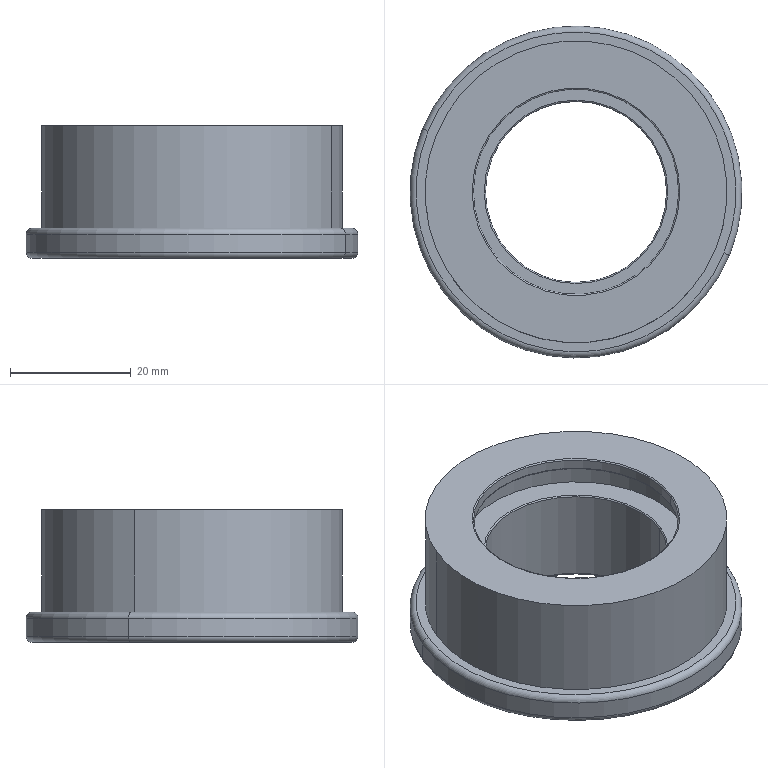Component | SolidWorks | Cylinder-1_GuideSleeve-1 | 1 solid | 27 faces | box 55 x 55 x 22 mm | volume 27518 mm3 | torus 12 | cylinder 10 | plane 5 | commonest cylinder face diameters 55 x2 50 x2 34 x2 38 x2 30 x2
build123d program:
from build123d import *

# Parameters (mm, degrees)
FILLET1_R = 1
FILLET2_R = 0.3
FILLET3_R = 0.2


with BuildPart() as part:
    # Sketch1 → Revolve1 (revolve)
    with BuildSketch(Plane.XY, mode=Mode.PRIVATE) as revolve1_sk:
        Polygon((0, 15), (16, 15), (16, 19), (20, 19), (20, 17), (22, 17), (22, 25), (5, 25), (5, 27.5), (0, 27.5), align=None)
    revolve(revolve1_sk.sketch.rotate(Axis((-21.725, 0, 0), (1, 0, 0)), 90), axis=Axis((-21.725, 0, 0), (1, 0, 0)))

    # Fillet1
    fillet1_edges = [part.edges().sort_by_distance(p)[0] for p in [
        (0, 0, -27.5),
        (5, 0, -27.5),
    ]]
    fillet(fillet1_edges, radius=FILLET1_R)

    # Fillet2
    fillet2_edges = [part.edges().sort_by_distance(p)[0] for p in [
        (0, 0, -15),
    ]]
    fillet(fillet2_edges, radius=FILLET2_R)

    # Fillet3
    fillet3_edges = [part.edges().sort_by_distance(p)[0] for p in [
        (16, 0, -15),
        (22, 0, -17),
        (20, 0, -17),
    ]]
    fillet(fillet3_edges, radius=FILLET3_R)


solid = part.part

# Placed as in the assembly
solid = solid.moved(Location((-180.557, 26.412, -199.351), (0, -90, 0)))
STEP:
#1=COLOUR_RGB('',0.7922,0.8196,0.9333);
#2=FILL_AREA_STYLE_COLOUR('',#1);
#3=FILL_AREA_STYLE('',(#2));
#4=SURFACE_STYLE_FILL_AREA(#3);
#5=SURFACE_SIDE_STYLE('',(#4));
#6=SURFACE_STYLE_USAGE(.BOTH.,#5);
#7=PRESENTATION_STYLE_ASSIGNMENT((#6));
#8=CARTESIAN_POINT('',(-6.563,0.8143,-7.226));
#9=VERTEX_POINT('',#8);
#10=CARTESIAN_POINT('',(-7.654,1.265,-7.226));
#11=VERTEX_POINT('',#10);
#12=CARTESIAN_POINT('',(-7.109,1.04,-7.226));
#13=DIRECTION('',(-0.,0.,1.));
#14=DIRECTION('',(-0.9242,0.3818,0.));
#15=AXIS2_PLACEMENT_3D('',#12,#13,#14);
#16=CIRCLE('',#15,0.5906);
#17=EDGE_CURVE('',#9,#11,#16,.T.);
#18=ORIENTED_EDGE('',*,*,#17,.F.);
#19=CARTESIAN_POINT('',(-6.555,0.8113,-7.219));
#20=VERTEX_POINT('',#19);
#21=CARTESIAN_POINT('',(-6.555,0.8113,-7.226));
#22=DIRECTION('',(0.3818,0.9242,-0.));
#23=DIRECTION('',(-0.9242,0.3818,0.));
#24=AXIS2_PLACEMENT_3D('',#21,#22,#23);
#25=CIRCLE('',#24,0.007874);
#26=EDGE_CURVE('',#9,#20,#25,.T.);
#27=ORIENTED_EDGE('',*,*,#26,.T.);
#28=CARTESIAN_POINT('',(-7.662,1.268,-7.219));
#29=VERTEX_POINT('',#28);
#30=CARTESIAN_POINT('',(-7.109,1.04,-7.219));
#31=DIRECTION('',(0.,-0.,-1.));
#32=DIRECTION('',(-0.9242,0.3818,0.));
#33=AXIS2_PLACEMENT_3D('',#30,#31,#32);
#34=CIRCLE('',#33,0.5984);
#35=EDGE_CURVE('',#29,#20,#34,.T.);
#36=ORIENTED_EDGE('',*,*,#35,.F.);
#37=CARTESIAN_POINT('',(-7.662,1.268,-7.226));
#38=DIRECTION('',(-0.3818,-0.9242,0.));
#39=DIRECTION('',(0.9242,-0.3818,0.));
#40=AXIS2_PLACEMENT_3D('',#37,#38,#39);
#41=CIRCLE('',#40,0.007874);
#42=EDGE_CURVE('',#11,#29,#41,.T.);
#43=ORIENTED_EDGE('',*,*,#42,.F.);
#44=EDGE_LOOP('',(#18,#27,#36,#43));
#45=FACE_OUTER_BOUND('',#44,.T.);
#46=CARTESIAN_POINT('',(-7.109,1.04,-7.226));
#47=DIRECTION('',(0.,-0.,-1.));
#48=DIRECTION('',(-0.9242,0.3818,-0.));
#49=AXIS2_PLACEMENT_3D('',#46,#47,#48);
#50=TOROIDAL_SURFACE('',#49,0.5984,0.007874);
#51=ADVANCED_FACE('',(#45),#50,.T.);
#52=CARTESIAN_POINT('',(-7.727,1.295,-7.053));
#53=VERTEX_POINT('',#52);
#54=CARTESIAN_POINT('',(-6.49,0.7843,-7.053));
#55=VERTEX_POINT('',#54);
#56=CARTESIAN_POINT('',(-7.109,1.04,-7.053));
#57=DIRECTION('',(0.,-0.,-1.));
#58=DIRECTION('',(0.9242,-0.3818,0.));
#59=AXIS2_PLACEMENT_3D('',#56,#57,#58);
#60=CIRCLE('',#59,0.6693);
#61=EDGE_CURVE('',#53,#55,#60,.T.);
#62=ORIENTED_EDGE('',*,*,#61,.F.);
#63=CARTESIAN_POINT('',(-7.734,1.298,-7.061));
#64=VERTEX_POINT('',#63);
#65=CARTESIAN_POINT('',(-7.734,1.298,-7.053));
#66=DIRECTION('',(0.3818,0.9242,-0.));
#67=DIRECTION('',(-0.9242,0.3818,0.));
#68=AXIS2_PLACEMENT_3D('',#65,#66,#67);
#69=CIRCLE('',#68,0.007874);
#70=EDGE_CURVE('',#53,#64,#69,.T.);
#71=ORIENTED_EDGE('',*,*,#70,.T.);
#72=CARTESIAN_POINT('',(-6.483,0.7813,-7.061));
#73=VERTEX_POINT('',#72);
#74=CARTESIAN_POINT('',(-7.109,1.04,-7.061));
#75=DIRECTION('',(-0.,0.,1.));
#76=DIRECTION('',(0.9242,-0.3818,0.));
#77=AXIS2_PLACEMENT_3D('',#74,#75,#76);
#78=CIRCLE('',#77,0.6772);
#79=EDGE_CURVE('',#73,#64,#78,.T.);
#80=ORIENTED_EDGE('',*,*,#79,.F.);
#81=CARTESIAN_POINT('',(-6.483,0.7813,-7.053));
#82=DIRECTION('',(-0.3818,-0.9242,0.));
#83=DIRECTION('',(0.9242,-0.3818,0.));
#84=AXIS2_PLACEMENT_3D('',#81,#82,#83);
#85=CIRCLE('',#84,0.007874);
#86=EDGE_CURVE('',#55,#73,#85,.T.);
#87=ORIENTED_EDGE('',*,*,#86,.F.);
#88=EDGE_LOOP('',(#62,#71,#80,#87));
#89=FACE_OUTER_BOUND('',#88,.T.);
#90=CARTESIAN_POINT('',(-7.109,1.04,-7.053));
#91=DIRECTION('',(-0.,0.,1.));
#92=DIRECTION('',(0.9242,-0.3818,0.));
#93=AXIS2_PLACEMENT_3D('',#90,#91,#92);
#94=TOROIDAL_SURFACE('',#93,0.6772,0.007874);
#95=ADVANCED_FACE('',(#89),#94,.T.);
#96=CARTESIAN_POINT('',(-6.49,0.7843,-6.99));
#97=VERTEX_POINT('',#96);
#98=CARTESIAN_POINT('',(-7.727,1.295,-6.99));
#99=VERTEX_POINT('',#98);
#100=CARTESIAN_POINT('',(-7.109,1.04,-6.99));
#101=DIRECTION('',(-0.,0.,1.));
#102=DIRECTION('',(-0.9242,0.3818,0.));
#103=AXIS2_PLACEMENT_3D('',#100,#101,#102);
#104=CIRCLE('',#103,0.6693);
#105=EDGE_CURVE('',#97,#99,#104,.T.);
#106=ORIENTED_EDGE('',*,*,#105,.F.);
#107=CARTESIAN_POINT('',(-6.483,0.7813,-6.982));
#108=VERTEX_POINT('',#107);
#109=CARTESIAN_POINT('',(-6.483,0.7813,-6.99));
#110=DIRECTION('',(0.3818,0.9242,-0.));
#111=DIRECTION('',(-0.9242,0.3818,0.));
#112=AXIS2_PLACEMENT_3D('',#109,#110,#111);
#113=CIRCLE('',#112,0.007874);
#114=EDGE_CURVE('',#97,#108,#113,.T.);
#115=ORIENTED_EDGE('',*,*,#114,.T.);
#116=CARTESIAN_POINT('',(-7.734,1.298,-6.982));
#117=VERTEX_POINT('',#116);
#118=CARTESIAN_POINT('',(-7.109,1.04,-6.982));
#119=DIRECTION('',(0.,-0.,-1.));
#120=DIRECTION('',(-0.9242,0.3818,0.));
#121=AXIS2_PLACEMENT_3D('',#118,#119,#120);
#122=CIRCLE('',#121,0.6772);
#123=EDGE_CURVE('',#117,#108,#122,.T.);
#124=ORIENTED_EDGE('',*,*,#123,.F.);
#125=CARTESIAN_POINT('',(-7.734,1.298,-6.99));
#126=DIRECTION('',(-0.3818,-0.9242,0.));
#127=DIRECTION('',(0.9242,-0.3818,0.));
#128=AXIS2_PLACEMENT_3D('',#125,#126,#127);
#129=CIRCLE('',#128,0.007874);
#130=EDGE_CURVE('',#99,#117,#129,.T.);
#131=ORIENTED_EDGE('',*,*,#130,.F.);
#132=EDGE_LOOP('',(#106,#115,#124,#131));
#133=FACE_OUTER_BOUND('',#132,.T.);
#134=CARTESIAN_POINT('',(-7.109,1.04,-6.99));
#135=DIRECTION('',(0.,-0.,-1.));
#136=DIRECTION('',(-0.9242,0.3818,-0.));
#137=AXIS2_PLACEMENT_3D('',#134,#135,#136);
#138=TOROIDAL_SURFACE('',#137,0.6772,0.007874);
#139=ADVANCED_FACE('',(#133),#138,.T.);
#140=CARTESIAN_POINT('',(-7.654,1.265,-7.837));
#141=VERTEX_POINT('',#140);
#142=CARTESIAN_POINT('',(-6.563,0.8143,-7.837));
#143=VERTEX_POINT('',#142);
#144=CARTESIAN_POINT('',(-7.109,1.04,-7.837));
#145=DIRECTION('',(0.,-0.,-1.));
#146=DIRECTION('',(0.9242,-0.3818,0.));
#147=AXIS2_PLACEMENT_3D('',#144,#145,#146);
#148=CIRCLE('',#147,0.5906);
#149=EDGE_CURVE('',#141,#143,#148,.T.);
#150=ORIENTED_EDGE('',*,*,#149,.F.);
#151=CARTESIAN_POINT('',(-7.665,1.27,-7.848));
#152=VERTEX_POINT('',#151);
#153=CARTESIAN_POINT('',(-7.665,1.27,-7.837));
#154=DIRECTION('',(0.3818,0.9242,-0.));
#155=DIRECTION('',(-0.9242,0.3818,0.));
#156=AXIS2_PLACEMENT_3D('',#153,#154,#155);
#157=CIRCLE('',#156,0.01181);
#158=EDGE_CURVE('',#141,#152,#157,.T.);
#159=ORIENTED_EDGE('',*,*,#158,.T.);
#160=CARTESIAN_POINT('',(-6.552,0.8098,-7.848));
#161=VERTEX_POINT('',#160);
#162=CARTESIAN_POINT('',(-7.109,1.04,-7.848));
#163=DIRECTION('',(-0.,0.,1.));
#164=DIRECTION('',(0.9242,-0.3818,0.));
#165=AXIS2_PLACEMENT_3D('',#162,#163,#164);
#166=CIRCLE('',#165,0.6024);
#167=EDGE_CURVE('',#161,#152,#166,.T.);
#168=ORIENTED_EDGE('',*,*,#167,.F.);
#169=CARTESIAN_POINT('',(-6.552,0.8098,-7.837));
#170=DIRECTION('',(-0.3818,-0.9242,0.));
#171=DIRECTION('',(0.9242,-0.3818,0.));
#172=AXIS2_PLACEMENT_3D('',#169,#170,#171);
#173=CIRCLE('',#172,0.01181);
#174=EDGE_CURVE('',#143,#161,#173,.T.);
#175=ORIENTED_EDGE('',*,*,#174,.F.);
#176=EDGE_LOOP('',(#150,#159,#168,#175));
#177=FACE_OUTER_BOUND('',#176,.T.);
#178=CARTESIAN_POINT('',(-7.109,1.04,-7.837));
#179=DIRECTION('',(-0.,0.,1.));
#180=DIRECTION('',(0.9242,-0.3818,0.));
#181=AXIS2_PLACEMENT_3D('',#178,#179,#180);
#182=TOROIDAL_SURFACE('',#181,0.6024,0.01181);
#183=ADVANCED_FACE('',(#177),#182,.T.);
#184=CARTESIAN_POINT('',(-6.144,0.6415,-7.652));
#185=VERTEX_POINT('',#184);
#186=CARTESIAN_POINT('',(-8.073,1.438,-7.652));
#187=VERTEX_POINT('',#186);
#188=CARTESIAN_POINT('',(-7.109,1.04,-7.652));
#189=DIRECTION('',(-0.,0.,1.));
#190=DIRECTION('',(-0.9242,0.3818,0.));
#191=AXIS2_PLACEMENT_3D('',#188,#189,#190);
#192=CIRCLE('',#191,1.043);
#193=EDGE_CURVE('',#185,#187,#192,.T.);
#194=ORIENTED_EDGE('',*,*,#193,.F.);
#195=CARTESIAN_POINT('',(-6.108,0.6264,-7.691));
#196=VERTEX_POINT('',#195);
#197=CARTESIAN_POINT('',(-6.144,0.6415,-7.691));
#198=DIRECTION('',(0.3818,0.9242,-0.));
#199=DIRECTION('',(-0.9242,0.3818,0.));
#200=AXIS2_PLACEMENT_3D('',#197,#198,#199);
#201=CIRCLE('',#200,0.03937);
#202=EDGE_CURVE('',#185,#196,#201,.T.);
#203=ORIENTED_EDGE('',*,*,#202,.T.);
#204=CARTESIAN_POINT('',(-8.109,1.453,-7.691));
#205=VERTEX_POINT('',#204);
#206=CARTESIAN_POINT('',(-7.109,1.04,-7.691));
#207=DIRECTION('',(0.,-0.,-1.));
#208=DIRECTION('',(-0.9242,0.3818,0.));
#209=AXIS2_PLACEMENT_3D('',#206,#207,#208);
#210=CIRCLE('',#209,1.083);
#211=EDGE_CURVE('',#205,#196,#210,.T.);
#212=ORIENTED_EDGE('',*,*,#211,.F.);
#213=CARTESIAN_POINT('',(-8.073,1.438,-7.691));
#214=DIRECTION('',(-0.3818,-0.9242,0.));
#215=DIRECTION('',(0.9242,-0.3818,0.));
#216=AXIS2_PLACEMENT_3D('',#213,#214,#215);
#217=CIRCLE('',#216,0.03937);
#218=EDGE_CURVE('',#187,#205,#217,.T.);
#219=ORIENTED_EDGE('',*,*,#218,.F.);
#220=EDGE_LOOP('',(#194,#203,#212,#219));
#221=FACE_OUTER_BOUND('',#220,.T.);
#222=CARTESIAN_POINT('',(-7.109,1.04,-7.691));
#223=DIRECTION('',(0.,-0.,-1.));
#224=DIRECTION('',(-0.9242,0.3818,-0.));
#225=AXIS2_PLACEMENT_3D('',#222,#223,#224);
#226=TOROIDAL_SURFACE('',#225,1.043,0.03937);
#227=ADVANCED_FACE('',(#221),#226,.T.);
#228=CARTESIAN_POINT('',(-8.073,1.438,-7.848));
#229=VERTEX_POINT('',#228);
#230=CARTESIAN_POINT('',(-6.144,0.6415,-7.848));
#231=VERTEX_POINT('',#230);
#232=CARTESIAN_POINT('',(-7.109,1.04,-7.848));
#233=DIRECTION('',(0.,-0.,-1.));
#234=DIRECTION('',(0.9242,-0.3818,0.));
#235=AXIS2_PLACEMENT_3D('',#232,#233,#234);
#236=CIRCLE('',#235,1.043);
#237=EDGE_CURVE('',#229,#231,#236,.T.);
#238=ORIENTED_EDGE('',*,*,#237,.F.);
#239=CARTESIAN_POINT('',(-8.109,1.453,-7.809));
#240=VERTEX_POINT('',#239);
#241=CARTESIAN_POINT('',(-8.073,1.438,-7.809));
#242=DIRECTION('',(0.3818,0.9242,-0.));
#243=DIRECTION('',(-0.9242,0.3818,0.));
#244=AXIS2_PLACEMENT_3D('',#241,#242,#243);
#245=CIRCLE('',#244,0.03937);
#246=EDGE_CURVE('',#229,#240,#245,.T.);
#247=ORIENTED_EDGE('',*,*,#246,.T.);
#248=CARTESIAN_POINT('',(-6.108,0.6264,-7.809));
#249=VERTEX_POINT('',#248);
#250=CARTESIAN_POINT('',(-7.109,1.04,-7.809));
#251=DIRECTION('',(-0.,0.,1.));
#252=DIRECTION('',(0.9242,-0.3818,0.));
#253=AXIS2_PLACEMENT_3D('',#250,#251,#252);
#254=CIRCLE('',#253,1.083);
#255=EDGE_CURVE('',#249,#240,#254,.T.);
#256=ORIENTED_EDGE('',*,*,#255,.F.);
#257=CARTESIAN_POINT('',(-6.144,0.6415,-7.809));
#258=DIRECTION('',(-0.3818,-0.9242,0.));
#259=DIRECTION('',(0.9242,-0.3818,0.));
#260=AXIS2_PLACEMENT_3D('',#257,#258,#259);
#261=CIRCLE('',#260,0.03937);
#262=EDGE_CURVE('',#231,#249,#261,.T.);
#263=ORIENTED_EDGE('',*,*,#262,.F.);
#264=EDGE_LOOP('',(#238,#247,#256,#263));
#265=FACE_OUTER_BOUND('',#264,.T.);
#266=CARTESIAN_POINT('',(-7.109,1.04,-7.809));
#267=DIRECTION('',(-0.,0.,1.));
#268=DIRECTION('',(0.9242,-0.3818,0.));
#269=AXIS2_PLACEMENT_3D('',#266,#267,#268);
#270=TOROIDAL_SURFACE('',#269,1.043,0.03937);
#271=ADVANCED_FACE('',(#265),#270,.T.);
#272=ORIENTED_EDGE('',*,*,#211,.T.);
#273=CARTESIAN_POINT('',(-6.108,0.6264,-8.704));
#274=DIRECTION('',(0.,-0.,-1.));
#275=VECTOR('',#274,39.37);
#276=LINE('',#273,#275);
#277=EDGE_CURVE('',#196,#249,#276,.T.);
#278=ORIENTED_EDGE('',*,*,#277,.T.);
#279=ORIENTED_EDGE('',*,*,#255,.T.);
#280=CARTESIAN_POINT('',(-8.109,1.453,-8.704));
#281=DIRECTION('',(0.,-0.,-1.));
#282=VECTOR('',#281,39.37);
#283=LINE('',#280,#282);
#284=EDGE_CURVE('',#205,#240,#283,.T.);
#285=ORIENTED_EDGE('',*,*,#284,.F.);
#286=EDGE_LOOP('',(#272,#278,#279,#285));
#287=FACE_OUTER_BOUND('',#286,.T.);
#288=CARTESIAN_POINT('',(-7.109,1.04,-8.704));
#289=DIRECTION('',(0.,-0.,-1.));
#290=DIRECTION('',(-0.9242,0.3818,0.));
#291=AXIS2_PLACEMENT_3D('',#288,#289,#290);
#292=CYLINDRICAL_SURFACE('',#291,1.083);
#293=ADVANCED_FACE('',(#287),#292,.T.);
#294=CARTESIAN_POINT('',(-8.018,1.416,-6.982));
#295=VERTEX_POINT('',#294);
#296=CARTESIAN_POINT('',(-6.199,0.664,-6.982));
#297=VERTEX_POINT('',#296);
#298=CARTESIAN_POINT('',(-7.109,1.04,-6.982));
#299=DIRECTION('',(0.,-0.,-1.));
#300=DIRECTION('',(-0.9242,0.3818,0.));
#301=AXIS2_PLACEMENT_3D('',#298,#299,#300);
#302=CIRCLE('',#301,0.9843);
#303=EDGE_CURVE('',#295,#297,#302,.T.);
#304=ORIENTED_EDGE('',*,*,#303,.T.);
#305=CARTESIAN_POINT('',(-6.199,0.664,-7.652));
#306=VERTEX_POINT('',#305);
#307=CARTESIAN_POINT('',(-6.199,0.664,-8.704));
#308=DIRECTION('',(0.,-0.,-1.));
#309=VECTOR('',#308,39.37);
#310=LINE('',#307,#309);
#311=EDGE_CURVE('',#297,#306,#310,.T.);
#312=ORIENTED_EDGE('',*,*,#311,.T.);
#313=CARTESIAN_POINT('',(-8.018,1.416,-7.652));
#314=VERTEX_POINT('',#313);
#315=CARTESIAN_POINT('',(-7.109,1.04,-7.652));
#316=DIRECTION('',(0.,-0.,-1.));
#317=DIRECTION('',(-0.9242,0.3818,0.));
#318=AXIS2_PLACEMENT_3D('',#315,#316,#317);
#319=CIRCLE('',#318,0.9843);
#320=EDGE_CURVE('',#314,#306,#319,.T.);
#321=ORIENTED_EDGE('',*,*,#320,.F.);
#322=CARTESIAN_POINT('',(-8.018,1.416,-8.704));
#323=DIRECTION('',(0.,-0.,-1.));
#324=VECTOR('',#323,39.37);
#325=LINE('',#322,#324);
#326=EDGE_CURVE('',#295,#314,#325,.T.);
#327=ORIENTED_EDGE('',*,*,#326,.F.);
#328=EDGE_LOOP('',(#304,#312,#321,#327));
#329=FACE_OUTER_BOUND('',#328,.T.);
#330=CARTESIAN_POINT('',(-7.109,1.04,-8.704));
#331=DIRECTION('',(0.,-0.,-1.));
#332=DIRECTION('',(-0.9242,0.3818,0.));
#333=AXIS2_PLACEMENT_3D('',#330,#331,#332);
#334=CYLINDRICAL_SURFACE('',#333,0.9843);
#335=ADVANCED_FACE('',(#329),#334,.T.);
#336=CARTESIAN_POINT('',(-7.109,1.04,-6.99));
#337=DIRECTION('',(-0.,0.,1.));
#338=DIRECTION('',(-0.9242,0.3818,0.));
#339=AXIS2_PLACEMENT_3D('',#336,#337,#338);
#340=CIRCLE('',#339,0.6693);
#341=EDGE_CURVE('',#99,#97,#340,.T.);
#342=ORIENTED_EDGE('',*,*,#341,.T.);
#343=CARTESIAN_POINT('',(-6.49,0.7843,-8.704));
#344=DIRECTION('',(0.,-0.,-1.));
#345=VECTOR('',#344,39.37);
#346=LINE('',#343,#345);
#347=EDGE_CURVE('',#97,#55,#346,.T.);
#348=ORIENTED_EDGE('',*,*,#347,.T.);
#349=CARTESIAN_POINT('',(-7.109,1.04,-7.053));
#350=DIRECTION('',(0.,-0.,-1.));
#351=DIRECTION('',(0.9242,-0.3818,0.));
#352=AXIS2_PLACEMENT_3D('',#349,#350,#351);
#353=CIRCLE('',#352,0.6693);
#354=EDGE_CURVE('',#55,#53,#353,.T.);
#355=ORIENTED_EDGE('',*,*,#354,.T.);
#356=CARTESIAN_POINT('',(-7.727,1.295,-8.704));
#357=DIRECTION('',(0.,-0.,-1.));
#358=VECTOR('',#357,39.37);
#359=LINE('',#356,#358);
#360=EDGE_CURVE('',#99,#53,#359,.T.);
#361=ORIENTED_EDGE('',*,*,#360,.F.);
#362=EDGE_LOOP('',(#342,#348,#355,#361));
#363=FACE_OUTER_BOUND('',#362,.T.);
#364=CARTESIAN_POINT('',(-7.109,1.04,-8.704));
#365=DIRECTION('',(0.,-0.,-1.));
#366=DIRECTION('',(-0.9242,0.3818,0.));
#367=AXIS2_PLACEMENT_3D('',#364,#365,#366);
#368=CYLINDRICAL_SURFACE('',#367,0.6693);
#369=ADVANCED_FACE('',(#363),#368,.F.);
#370=CARTESIAN_POINT('',(-6.417,0.7542,-7.061));
#371=VERTEX_POINT('',#370);
#372=CARTESIAN_POINT('',(-7.8,1.325,-7.061));
#373=VERTEX_POINT('',#372);
#374=CARTESIAN_POINT('',(-7.109,1.04,-7.061));
#375=DIRECTION('',(0.,-0.,-1.));
#376=DIRECTION('',(-0.9242,0.3818,0.));
#377=AXIS2_PLACEMENT_3D('',#374,#375,#376);
#378=CIRCLE('',#377,0.748);
#379=EDGE_CURVE('',#371,#373,#378,.T.);
#380=ORIENTED_EDGE('',*,*,#379,.F.);
#381=CARTESIAN_POINT('',(-6.417,0.7542,-7.219));
#382=VERTEX_POINT('',#381);
#383=CARTESIAN_POINT('',(-6.417,0.7542,-8.704));
#384=DIRECTION('',(0.,-0.,-1.));
#385=VECTOR('',#384,39.37);
#386=LINE('',#383,#385);
#387=EDGE_CURVE('',#371,#382,#386,.T.);
#388=ORIENTED_EDGE('',*,*,#387,.T.);
#389=CARTESIAN_POINT('',(-7.8,1.325,-7.219));
#390=VERTEX_POINT('',#389);
#391=CARTESIAN_POINT('',(-7.109,1.04,-7.219));
#392=DIRECTION('',(0.,-0.,-1.));
#393=DIRECTION('',(-0.9242,0.3818,0.));
#394=AXIS2_PLACEMENT_3D('',#391,#392,#393);
#395=CIRCLE('',#394,0.748);
#396=EDGE_CURVE('',#382,#390,#395,.T.);
#397=ORIENTED_EDGE('',*,*,#396,.T.);
#398=CARTESIAN_POINT('',(-7.8,1.325,-8.704));
#399=DIRECTION('',(0.,-0.,-1.));
#400=VECTOR('',#399,39.37);
#401=LINE('',#398,#400);
#402=EDGE_CURVE('',#373,#390,#401,.T.);
#403=ORIENTED_EDGE('',*,*,#402,.F.);
#404=EDGE_LOOP('',(#380,#388,#397,#403));
#405=FACE_OUTER_BOUND('',#404,.T.);
#406=CARTESIAN_POINT('',(-7.109,1.04,-8.704));
#407=DIRECTION('',(0.,-0.,-1.));
#408=DIRECTION('',(-0.9242,0.3818,0.));
#409=AXIS2_PLACEMENT_3D('',#406,#407,#408);
#410=CYLINDRICAL_SURFACE('',#409,0.748);
#411=ADVANCED_FACE('',(#405),#410,.F.);
#412=CARTESIAN_POINT('',(-7.109,1.04,-7.226));
#413=DIRECTION('',(-0.,0.,1.));
#414=DIRECTION('',(-0.9242,0.3818,0.));
#415=AXIS2_PLACEMENT_3D('',#412,#413,#414);
#416=CIRCLE('',#415,0.5906);
#417=EDGE_CURVE('',#11,#9,#416,.T.);
#418=ORIENTED_EDGE('',*,*,#417,.T.);
#419=CARTESIAN_POINT('',(-6.563,0.8143,-8.704));
#420=DIRECTION('',(0.,-0.,-1.));
#421=VECTOR('',#420,39.37);
#422=LINE('',#419,#421);
#423=EDGE_CURVE('',#9,#143,#422,.T.);
#424=ORIENTED_EDGE('',*,*,#423,.T.);
#425=CARTESIAN_POINT('',(-7.109,1.04,-7.837));
#426=DIRECTION('',(0.,-0.,-1.));
#427=DIRECTION('',(0.9242,-0.3818,0.));
#428=AXIS2_PLACEMENT_3D('',#425,#426,#427);
#429=CIRCLE('',#428,0.5906);
#430=EDGE_CURVE('',#143,#141,#429,.T.);
#431=ORIENTED_EDGE('',*,*,#430,.T.);
#432=CARTESIAN_POINT('',(-7.654,1.265,-8.704));
#433=DIRECTION('',(0.,-0.,-1.));
#434=VECTOR('',#433,39.37);
#435=LINE('',#432,#434);
#436=EDGE_CURVE('',#11,#141,#435,.T.);
#437=ORIENTED_EDGE('',*,*,#436,.F.);
#438=EDGE_LOOP('',(#418,#424,#431,#437));
#439=FACE_OUTER_BOUND('',#438,.T.);
#440=CARTESIAN_POINT('',(-7.109,1.04,-8.704));
#441=DIRECTION('',(0.,-0.,-1.));
#442=DIRECTION('',(-0.9242,0.3818,0.));
#443=AXIS2_PLACEMENT_3D('',#440,#441,#442);
#444=CYLINDRICAL_SURFACE('',#443,0.5906);
#445=ADVANCED_FACE('',(#439),#444,.F.);
#446=ORIENTED_EDGE('',*,*,#167,.T.);
#447=CARTESIAN_POINT('',(-7.109,1.04,-7.848));
#448=DIRECTION('',(-0.,0.,1.));
#449=DIRECTION('',(0.9242,-0.3818,0.));
#450=AXIS2_PLACEMENT_3D('',#447,#448,#449);
#451=CIRCLE('',#450,0.6024);
#452=EDGE_CURVE('',#152,#161,#451,.T.);
#453=ORIENTED_EDGE('',*,*,#452,.T.);
#454=EDGE_LOOP('',(#446,#453));
#455=FACE_BOUND('',#454,.T.);
#456=CARTESIAN_POINT('',(-7.109,1.04,-7.848));
#457=DIRECTION('',(0.,-0.,-1.));
#458=DIRECTION('',(0.9242,-0.3818,0.));
#459=AXIS2_PLACEMENT_3D('',#456,#457,#458);
#460=CIRCLE('',#459,1.043);
#461=EDGE_CURVE('',#231,#229,#460,.T.);
#462=ORIENTED_EDGE('',*,*,#461,.T.);
#463=ORIENTED_EDGE('',*,*,#237,.T.);
#464=EDGE_LOOP('',(#462,#463));
#465=FACE_OUTER_BOUND('',#464,.T.);
#466=CARTESIAN_POINT('',(-6.695,2.04,-7.848));
#467=DIRECTION('',(-0.,0.,1.));
#468=DIRECTION('',(0.9242,-0.3818,0.));
#469=AXIS2_PLACEMENT_3D('',#466,#467,#468);
#470=PLANE('',#469);
#471=ADVANCED_FACE('',(#455,#465),#470,.F.);
#472=ORIENTED_EDGE('',*,*,#423,.F.);
#473=ORIENTED_EDGE('',*,*,#17,.T.);
#474=ORIENTED_EDGE('',*,*,#436,.T.);
#475=ORIENTED_EDGE('',*,*,#149,.T.);
#476=EDGE_LOOP('',(#472,#473,#474,#475));
#477=FACE_OUTER_BOUND('',#476,.T.);
#478=CARTESIAN_POINT('',(-7.109,1.04,-8.704));
#479=DIRECTION('',(0.,-0.,-1.));
#480=DIRECTION('',(-0.9242,0.3818,0.));
#481=AXIS2_PLACEMENT_3D('',#478,#479,#480);
#482=CYLINDRICAL_SURFACE('',#481,0.5906);
#483=ADVANCED_FACE('',(#477),#482,.F.);
#484=ORIENTED_EDGE('',*,*,#35,.T.);
#485=CARTESIAN_POINT('',(-7.109,1.04,-7.219));
#486=DIRECTION('',(0.,-0.,-1.));
#487=DIRECTION('',(-0.9242,0.3818,0.));
#488=AXIS2_PLACEMENT_3D('',#485,#486,#487);
#489=CIRCLE('',#488,0.5984);
#490=EDGE_CURVE('',#20,#29,#489,.T.);
#491=ORIENTED_EDGE('',*,*,#490,.T.);
#492=EDGE_LOOP('',(#484,#491));
#493=FACE_BOUND('',#492,.T.);
#494=CARTESIAN_POINT('',(-7.109,1.04,-7.219));
#495=DIRECTION('',(0.,-0.,-1.));
#496=DIRECTION('',(-0.9242,0.3818,0.));
#497=AXIS2_PLACEMENT_3D('',#494,#495,#496);
#498=CIRCLE('',#497,0.748);
#499=EDGE_CURVE('',#390,#382,#498,.T.);
#500=ORIENTED_EDGE('',*,*,#499,.F.);
#501=ORIENTED_EDGE('',*,*,#396,.F.);
#502=EDGE_LOOP('',(#500,#501));
#503=FACE_OUTER_BOUND('',#502,.T.);
#504=CARTESIAN_POINT('',(-6.883,1.586,-7.219));
#505=DIRECTION('',(0.,-0.,-1.));
#506=DIRECTION('',(-0.9242,0.3818,-0.));
#507=AXIS2_PLACEMENT_3D('',#504,#505,#506);
#508=PLANE('',#507);
#509=ADVANCED_FACE('',(#493,#503),#508,.F.);
#510=ORIENTED_EDGE('',*,*,#387,.F.);
#511=CARTESIAN_POINT('',(-7.109,1.04,-7.061));
#512=DIRECTION('',(0.,-0.,-1.));
#513=DIRECTION('',(-0.9242,0.3818,0.));
#514=AXIS2_PLACEMENT_3D('',#511,#512,#513);
#515=CIRCLE('',#514,0.748);
#516=EDGE_CURVE('',#373,#371,#515,.T.);
#517=ORIENTED_EDGE('',*,*,#516,.F.);
#518=ORIENTED_EDGE('',*,*,#402,.T.);
#519=ORIENTED_EDGE('',*,*,#499,.T.);
#520=EDGE_LOOP('',(#510,#517,#518,#519));
#521=FACE_OUTER_BOUND('',#520,.T.);
#522=CARTESIAN_POINT('',(-7.109,1.04,-8.704));
#523=DIRECTION('',(0.,-0.,-1.));
#524=DIRECTION('',(-0.9242,0.3818,0.));
#525=AXIS2_PLACEMENT_3D('',#522,#523,#524);
#526=CYLINDRICAL_SURFACE('',#525,0.748);
#527=ADVANCED_FACE('',(#521),#526,.F.);
#528=ORIENTED_EDGE('',*,*,#79,.T.);
#529=CARTESIAN_POINT('',(-7.109,1.04,-7.061));
#530=DIRECTION('',(-0.,0.,1.));
#531=DIRECTION('',(0.9242,-0.3818,0.));
#532=AXIS2_PLACEMENT_3D('',#529,#530,#531);
#533=CIRCLE('',#532,0.6772);
#534=EDGE_CURVE('',#64,#73,#533,.T.);
#535=ORIENTED_EDGE('',*,*,#534,.T.);
#536=EDGE_LOOP('',(#528,#535));
#537=FACE_BOUND('',#536,.T.);
#538=ORIENTED_EDGE('',*,*,#516,.T.);
#539=ORIENTED_EDGE('',*,*,#379,.T.);
#540=EDGE_LOOP('',(#538,#539));
#541=FACE_OUTER_BOUND('',#540,.T.);
#542=CARTESIAN_POINT('',(-6.823,1.731,-7.061));
#543=DIRECTION('',(-0.,0.,1.));
#544=DIRECTION('',(0.9242,-0.3818,0.));
#545=AXIS2_PLACEMENT_3D('',#542,#543,#544);
#546=PLANE('',#545);
#547=ADVANCED_FACE('',(#537,#541),#546,.F.);
#548=ORIENTED_EDGE('',*,*,#347,.F.);
#549=ORIENTED_EDGE('',*,*,#105,.T.);
#550=ORIENTED_EDGE('',*,*,#360,.T.);
#551=ORIENTED_EDGE('',*,*,#61,.T.);
#552=EDGE_LOOP('',(#548,#549,#550,#551));
#553=FACE_OUTER_BOUND('',#552,.T.);
#554=CARTESIAN_POINT('',(-7.109,1.04,-8.704));
#555=DIRECTION('',(0.,-0.,-1.));
#556=DIRECTION('',(-0.9242,0.3818,0.));
#557=AXIS2_PLACEMENT_3D('',#554,#555,#556);
#558=CYLINDRICAL_SURFACE('',#557,0.6693);
#559=ADVANCED_FACE('',(#553),#558,.F.);
#560=ORIENTED_EDGE('',*,*,#123,.T.);
#561=CARTESIAN_POINT('',(-7.109,1.04,-6.982));
#562=DIRECTION('',(0.,-0.,-1.));
#563=DIRECTION('',(-0.9242,0.3818,0.));
#564=AXIS2_PLACEMENT_3D('',#561,#562,#563);
#565=CIRCLE('',#564,0.6772);
#566=EDGE_CURVE('',#108,#117,#565,.T.);
#567=ORIENTED_EDGE('',*,*,#566,.T.);
#568=EDGE_LOOP('',(#560,#567));
#569=FACE_BOUND('',#568,.T.);
#570=ORIENTED_EDGE('',*,*,#303,.F.);
#571=CARTESIAN_POINT('',(-7.109,1.04,-6.982));
#572=DIRECTION('',(0.,-0.,-1.));
#573=DIRECTION('',(-0.9242,0.3818,0.));
#574=AXIS2_PLACEMENT_3D('',#571,#572,#573);
#575=CIRCLE('',#574,0.9843);
#576=EDGE_CURVE('',#297,#295,#575,.T.);
#577=ORIENTED_EDGE('',*,*,#576,.F.);
#578=EDGE_LOOP('',(#570,#577));
#579=FACE_OUTER_BOUND('',#578,.T.);
#580=CARTESIAN_POINT('',(-6.853,1.658,-6.982));
#581=DIRECTION('',(0.,-0.,-1.));
#582=DIRECTION('',(-0.9242,0.3818,-0.));
#583=AXIS2_PLACEMENT_3D('',#580,#581,#582);
#584=PLANE('',#583);
#585=ADVANCED_FACE('',(#569,#579),#584,.F.);
#586=ORIENTED_EDGE('',*,*,#311,.F.);
#587=ORIENTED_EDGE('',*,*,#576,.T.);
#588=ORIENTED_EDGE('',*,*,#326,.T.);
#589=CARTESIAN_POINT('',(-7.109,1.04,-7.652));
#590=DIRECTION('',(0.,-0.,-1.));
#591=DIRECTION('',(-0.9242,0.3818,0.));
#592=AXIS2_PLACEMENT_3D('',#589,#590,#591);
#593=CIRCLE('',#592,0.9843);
#594=EDGE_CURVE('',#306,#314,#593,.T.);
#595=ORIENTED_EDGE('',*,*,#594,.F.);
#596=EDGE_LOOP('',(#586,#587,#588,#595));
#597=FACE_OUTER_BOUND('',#596,.T.);
#598=CARTESIAN_POINT('',(-7.109,1.04,-8.704));
#599=DIRECTION('',(0.,-0.,-1.));
#600=DIRECTION('',(-0.9242,0.3818,0.));
#601=AXIS2_PLACEMENT_3D('',#598,#599,#600);
#602=CYLINDRICAL_SURFACE('',#601,0.9843);
#603=ADVANCED_FACE('',(#597),#602,.T.);
#604=CARTESIAN_POINT('',(-7.109,1.04,-7.652));
#605=DIRECTION('',(-0.,0.,1.));
#606=DIRECTION('',(-0.9242,0.3818,0.));
#607=AXIS2_PLACEMENT_3D('',#604,#605,#606);
#608=CIRCLE('',#607,1.043);
#609=EDGE_CURVE('',#187,#185,#608,.T.);
#610=ORIENTED_EDGE('',*,*,#609,.T.);
#611=ORIENTED_EDGE('',*,*,#193,.T.);
#612=EDGE_LOOP('',(#610,#611));
#613=FACE_OUTER_BOUND('',#612,.T.);
#614=ORIENTED_EDGE('',*,*,#320,.T.);
#615=ORIENTED_EDGE('',*,*,#594,.T.);
#616=EDGE_LOOP('',(#614,#615));
#617=FACE_BOUND('',#616,.T.);
#618=CARTESIAN_POINT('',(-6.733,1.95,-7.652));
#619=DIRECTION('',(0.,-0.,-1.));
#620=DIRECTION('',(-0.9242,0.3818,-0.));
#621=AXIS2_PLACEMENT_3D('',#618,#619,#620);
#622=PLANE('',#621);
#623=ADVANCED_FACE('',(#613,#617),#622,.F.);
#624=ORIENTED_EDGE('',*,*,#277,.F.);
#625=CARTESIAN_POINT('',(-7.109,1.04,-7.691));
#626=DIRECTION('',(0.,-0.,-1.));
#627=DIRECTION('',(-0.9242,0.3818,0.));
#628=AXIS2_PLACEMENT_3D('',#625,#626,#627);
#629=CIRCLE('',#628,1.083);
#630=EDGE_CURVE('',#196,#205,#629,.T.);
#631=ORIENTED_EDGE('',*,*,#630,.T.);
#632=ORIENTED_EDGE('',*,*,#284,.T.);
#633=CARTESIAN_POINT('',(-7.109,1.04,-7.809));
#634=DIRECTION('',(-0.,0.,1.));
#635=DIRECTION('',(0.9242,-0.3818,0.));
#636=AXIS2_PLACEMENT_3D('',#633,#634,#635);
#637=CIRCLE('',#636,1.083);
#638=EDGE_CURVE('',#240,#249,#637,.T.);
#639=ORIENTED_EDGE('',*,*,#638,.T.);
#640=EDGE_LOOP('',(#624,#631,#632,#639));
#641=FACE_OUTER_BOUND('',#640,.T.);
#642=CARTESIAN_POINT('',(-7.109,1.04,-8.704));
#643=DIRECTION('',(0.,-0.,-1.));
#644=DIRECTION('',(-0.9242,0.3818,0.));
#645=AXIS2_PLACEMENT_3D('',#642,#643,#644);
#646=CYLINDRICAL_SURFACE('',#645,1.083);
#647=ADVANCED_FACE('',(#641),#646,.T.);
#648=ORIENTED_EDGE('',*,*,#246,.F.);
#649=ORIENTED_EDGE('',*,*,#461,.F.);
#650=ORIENTED_EDGE('',*,*,#262,.T.);
#651=ORIENTED_EDGE('',*,*,#638,.F.);
#652=EDGE_LOOP('',(#648,#649,#650,#651));
#653=FACE_OUTER_BOUND('',#652,.T.);
#654=CARTESIAN_POINT('',(-7.109,1.04,-7.809));
#655=DIRECTION('',(-0.,0.,1.));
#656=DIRECTION('',(0.9242,-0.3818,0.));
#657=AXIS2_PLACEMENT_3D('',#654,#655,#656);
#658=TOROIDAL_SURFACE('',#657,1.043,0.03937);
#659=ADVANCED_FACE('',(#653),#658,.T.);
#660=ORIENTED_EDGE('',*,*,#202,.F.);
#661=ORIENTED_EDGE('',*,*,#609,.F.);
#662=ORIENTED_EDGE('',*,*,#218,.T.);
#663=ORIENTED_EDGE('',*,*,#630,.F.);
#664=EDGE_LOOP('',(#660,#661,#662,#663));
#665=FACE_OUTER_BOUND('',#664,.T.);
#666=CARTESIAN_POINT('',(-7.109,1.04,-7.691));
#667=DIRECTION('',(0.,-0.,-1.));
#668=DIRECTION('',(-0.9242,0.3818,-0.));
#669=AXIS2_PLACEMENT_3D('',#666,#667,#668);
#670=TOROIDAL_SURFACE('',#669,1.043,0.03937);
#671=ADVANCED_FACE('',(#665),#670,.T.);
#672=ORIENTED_EDGE('',*,*,#158,.F.);
#673=ORIENTED_EDGE('',*,*,#430,.F.);
#674=ORIENTED_EDGE('',*,*,#174,.T.);
#675=ORIENTED_EDGE('',*,*,#452,.F.);
#676=EDGE_LOOP('',(#672,#673,#674,#675));
#677=FACE_OUTER_BOUND('',#676,.T.);
#678=CARTESIAN_POINT('',(-7.109,1.04,-7.837));
#679=DIRECTION('',(-0.,0.,1.));
#680=DIRECTION('',(0.9242,-0.3818,0.));
#681=AXIS2_PLACEMENT_3D('',#678,#679,#680);
#682=TOROIDAL_SURFACE('',#681,0.6024,0.01181);
#683=ADVANCED_FACE('',(#677),#682,.T.);
#684=ORIENTED_EDGE('',*,*,#114,.F.);
#685=ORIENTED_EDGE('',*,*,#341,.F.);
#686=ORIENTED_EDGE('',*,*,#130,.T.);
#687=ORIENTED_EDGE('',*,*,#566,.F.);
#688=EDGE_LOOP('',(#684,#685,#686,#687));
#689=FACE_OUTER_BOUND('',#688,.T.);
#690=CARTESIAN_POINT('',(-7.109,1.04,-6.99));
#691=DIRECTION('',(0.,-0.,-1.));
#692=DIRECTION('',(-0.9242,0.3818,-0.));
#693=AXIS2_PLACEMENT_3D('',#690,#691,#692);
#694=TOROIDAL_SURFACE('',#693,0.6772,0.007874);
#695=ADVANCED_FACE('',(#689),#694,.T.);
#696=ORIENTED_EDGE('',*,*,#70,.F.);
#697=ORIENTED_EDGE('',*,*,#354,.F.);
#698=ORIENTED_EDGE('',*,*,#86,.T.);
#699=ORIENTED_EDGE('',*,*,#534,.F.);
#700=EDGE_LOOP('',(#696,#697,#698,#699));
#701=FACE_OUTER_BOUND('',#700,.T.);
#702=CARTESIAN_POINT('',(-7.109,1.04,-7.053));
#703=DIRECTION('',(-0.,0.,1.));
#704=DIRECTION('',(0.9242,-0.3818,0.));
#705=AXIS2_PLACEMENT_3D('',#702,#703,#704);
#706=TOROIDAL_SURFACE('',#705,0.6772,0.007874);
#707=ADVANCED_FACE('',(#701),#706,.T.);
#708=ORIENTED_EDGE('',*,*,#26,.F.);
#709=ORIENTED_EDGE('',*,*,#417,.F.);
#710=ORIENTED_EDGE('',*,*,#42,.T.);
#711=ORIENTED_EDGE('',*,*,#490,.F.);
#712=EDGE_LOOP('',(#708,#709,#710,#711));
#713=FACE_OUTER_BOUND('',#712,.T.);
#714=CARTESIAN_POINT('',(-7.109,1.04,-7.226));
#715=DIRECTION('',(0.,-0.,-1.));
#716=DIRECTION('',(-0.9242,0.3818,-0.));
#717=AXIS2_PLACEMENT_3D('',#714,#715,#716);
#718=TOROIDAL_SURFACE('',#717,0.5984,0.007874);
#719=ADVANCED_FACE('',(#713),#718,.T.);
#720=CLOSED_SHELL('',(#51,#95,#139,#183,#227,#271,#293,#335,#369,#411,#445,#471,#483,#509,#527,#547,#559,#585,#603,#623,#647,#659,#671,#683,#695,#707,#719));
#721=MANIFOLD_SOLID_BREP('',#720);
#722=STYLED_ITEM('',(#7),#721);
#723=(LENGTH_UNIT()NAMED_UNIT(*)SI_UNIT($,.METRE.));
#724=LENGTH_MEASURE_WITH_UNIT(LENGTH_MEASURE(0.0254),#723);
#725=DIMENSIONAL_EXPONENTS(1.,0.,0.,0.,0.,0.,0.);
#726=(CONVERSION_BASED_UNIT('',#724)LENGTH_UNIT()NAMED_UNIT(#725));
#727=UNCERTAINTY_MEASURE_WITH_UNIT(LENGTH_MEASURE(0.00001),#726,'','');
#728=(NAMED_UNIT(*)PLANE_ANGLE_UNIT()SI_UNIT($,.RADIAN.));
#729=(NAMED_UNIT(*)SI_UNIT($,.STERADIAN.)SOLID_ANGLE_UNIT());
#730=(GEOMETRIC_REPRESENTATION_CONTEXT(3)GLOBAL_UNCERTAINTY_ASSIGNED_CONTEXT((#727))GLOBAL_UNIT_ASSIGNED_CONTEXT((#726,#728,#729))REPRESENTATION_CONTEXT('',''));
#731=MECHANICAL_DESIGN_GEOMETRIC_PRESENTATION_REPRESENTATION('',(#722),#730);
#732=PRESENTATION_LAYER_ASSIGNMENT('','',(#722));
#733=CARTESIAN_POINT('',(0.,0.,0.));
#734=DIRECTION('',(0.,0.,1.));
#735=DIRECTION('',(1.,0.,0.));
#736=AXIS2_PLACEMENT_3D('',#733,#734,#735);
#737=(LENGTH_UNIT()NAMED_UNIT(*)SI_UNIT($,.METRE.));
#738=LENGTH_MEASURE_WITH_UNIT(LENGTH_MEASURE(0.0254),#737);
#739=DIMENSIONAL_EXPONENTS(1.,0.,0.,0.,0.,0.,0.);
#740=(CONVERSION_BASED_UNIT('',#738)LENGTH_UNIT()NAMED_UNIT(#739));
#741=UNCERTAINTY_MEASURE_WITH_UNIT(LENGTH_MEASURE(0.00001),#740,'','');
#742=(NAMED_UNIT(*)PLANE_ANGLE_UNIT()SI_UNIT($,.RADIAN.));
#743=(NAMED_UNIT(*)SI_UNIT($,.STERADIAN.)SOLID_ANGLE_UNIT());
#744=(GEOMETRIC_REPRESENTATION_CONTEXT(3)GLOBAL_UNCERTAINTY_ASSIGNED_CONTEXT((#741))GLOBAL_UNIT_ASSIGNED_CONTEXT((#740,#742,#743))REPRESENTATION_CONTEXT('',''));
#745=ADVANCED_BREP_SHAPE_REPRESENTATION('',(#721,#736),#744);